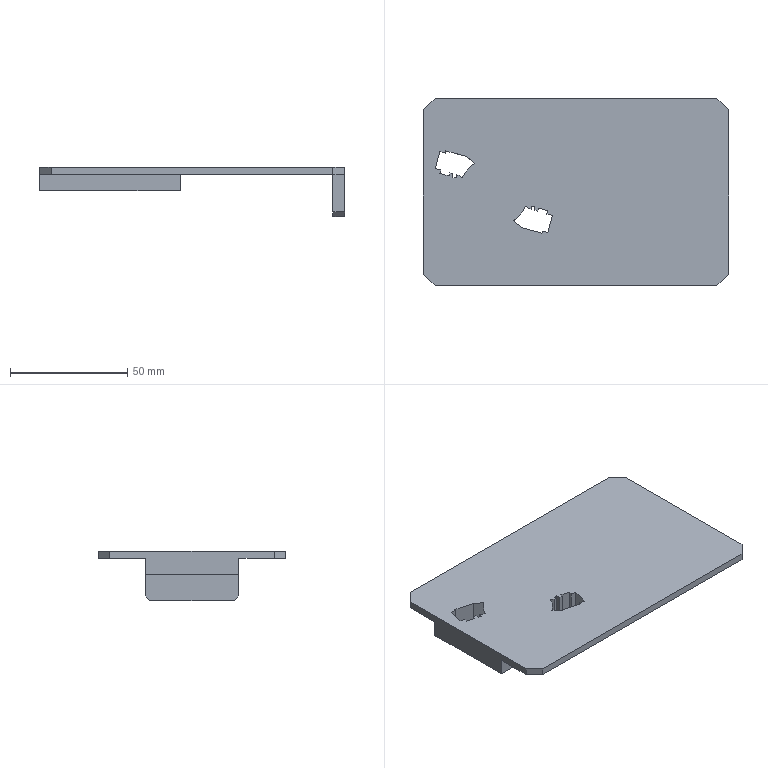Component | SolidWorks | 2023-12-12-27-1 | 1 solid | 52 faces | box 130 x 80 x 21 mm | volume 48991 mm3 | plane 50 | cylinder 2 | commonest cylinder face diameters 29.56 x2 | material S45C
build123d program:
from build123d import *

# Parameters (mm, degrees)
SKETCH1_R           = 14.78
BOSS_EXTRUDE1_DEPTH = 10
SKETCH2_W           = 60
SKETCH2_H           = 80
BOSS_EXTRUDE2_DEPTH = 10
CUT_EXTRUDE1_DEPTH  = 51.99
MOVE_FACE1_BY       = 70
SKETCH4_W           = 7
SKETCH4_H           = 20
CUT_EXTRUDE2_DEPTH  = 137.382
CHAMFER1_SIZE       = 5
SKETCH5_W           = 65
SKETCH5_H           = 40
CUT_EXTRUDE3_DEPTH  = 7
MOVE_FACE2_BY       = 11
CHAMFER2_SIZE       = 2


with BuildPart() as part:
    # Sketch1 → Boss-Extrude1 (new body)
    with BuildSketch(Plane.XY):
        Circle(SKETCH1_R)
    extrude(amount=BOSS_EXTRUDE1_DEPTH)

    # Sketch2 → Boss-Extrude2 (add)
    with BuildSketch(Plane(origin=(0, 0, 0), x_dir=(-1, 0, 0), z_dir=(0, 0, -1))):
        Rectangle(SKETCH2_W, SKETCH2_H)
    extrude(amount=-BOSS_EXTRUDE2_DEPTH)

    # Sketch3 → Cut-Extrude1 (cut, through all)
    with BuildSketch(Plane.XY.offset(10)):
        with BuildLine():
            Line((-11.655, 15.132), (-8.242, 12.268))
            ThreePointArc((-8.242, 12.268), (-11.322, 9.5), (-13.513, 5.987))
            Line((-13.513, 5.987), (-14.809, 7.074))
            Line((-14.809, 7.074), (-15.9, 7.366))
            Line((-15.9, 7.366), (-15.9, 6))
            Line((-15.9, 6), (-17.5, 6))
            Line((-17.5, 6), (-17.5, 7.795))
            Line((-17.5, 7.795), (-18.735, 8.126))
            Line((-18.735, 8.126), (-19.072, 6.87))
            Line((-19.072, 6.87), (-23.004, 7.924))
            Line((-23.004, 7.924), (-22.616, 9.373))
            Line((-22.616, 9.373), (-24.934, 9.994))
            Line((-24.934, 9.994), (-22.993, 17.238))
            Line((-22.993, 17.238), (-20.675, 16.617))
            Line((-20.675, 16.617), (-20.442, 17.487))
            Line((-20.442, 17.487), (-18.5, 16.966))
            Line((-18.5, 16.966), (-11.655, 15.132))
        make_face()
        with BuildLine():
            Line((17.5, -7.795), (18.735, -8.126))
            Line((18.735, -8.126), (19.072, -6.87))
            Line((19.072, -6.87), (23.004, -7.924))
            Line((23.004, -7.924), (22.616, -9.373))
            Line((22.616, -9.373), (24.934, -9.994))
            Line((24.934, -9.994), (22.993, -17.238))
            Line((22.993, -17.238), (20.675, -16.617))
            Line((20.675, -16.617), (20.442, -17.487))
            Line((20.442, -17.487), (18.5, -16.966))
            Line((18.5, -16.966), (11.655, -15.132))
            Line((11.655, -15.132), (8.242, -12.268))
            ThreePointArc((8.242, -12.268), (11.322, -9.5), (13.513, -5.987))
            Line((13.513, -5.987), (14.809, -7.074))
            Line((14.809, -7.074), (15.9, -7.366))
            Line((15.9, -7.366), (15.9, -6))
            Line((15.9, -6), (17.5, -6))
            Line((17.5, -6), (17.5, -7.795))
        make_face()
    extrude(amount=-CUT_EXTRUDE1_DEPTH, mode=Mode.SUBTRACT)

    # Move Face1: a face moved outward by 70.0
    extrude(part.faces().sort_by_distance((-30, 0, 5))[0], amount=MOVE_FACE1_BY, dir=(-1, 0, 0))

    # Sketch4 → Cut-Extrude2 (cut, through all)
    with BuildSketch(Plane(origin=(30, 0, 0), x_dir=(0, 0, -1), z_dir=(1, 0, 0))):
        with Locations((-3.5, -30)):
            Rectangle(SKETCH4_W, SKETCH4_H)
        with Locations((-3.5, 30)):
            Rectangle(SKETCH4_W, SKETCH4_H)
    extrude(amount=-CUT_EXTRUDE2_DEPTH, mode=Mode.SUBTRACT)

    # Chamfer1
    chamfer1_edges = [part.edges().sort_by_distance(p)[0] for p in [
        (30, 40, 8.5),
        (30, -40, 8.5),
        (-100, -40, 8.5),
        (-100, 40, 8.5),
    ]]
    chamfer(chamfer1_edges, length=CHAMFER1_SIZE)

    # Sketch5 → Cut-Extrude3 (cut)
    with BuildSketch(Plane(origin=(0, 0, 0), x_dir=(-1, 0, 0), z_dir=(0, 0, -1))):
        with Locations((62.5, 0)):
            Rectangle(SKETCH5_W, SKETCH5_H)
    extrude(amount=-CUT_EXTRUDE3_DEPTH, mode=Mode.SUBTRACT)

    # Move Face2: a face moved outward by 11.0
    extrude(part.faces().sort_by_distance((-97.5, 0, 0))[0], amount=MOVE_FACE2_BY, dir=(0, 0, -1))

    # Chamfer2
    chamfer2_edges = [part.edges().sort_by_distance(p)[0] for p in [
        (-97.5, -20, -11),
        (-97.5, 20, -11),
    ]]
    chamfer(chamfer2_edges, length=CHAMFER2_SIZE)


solid = part.part

# Placed as in the assembly
solid = solid.moved(Location((-68.778, -2.867, 84), (0, 0, 180)))